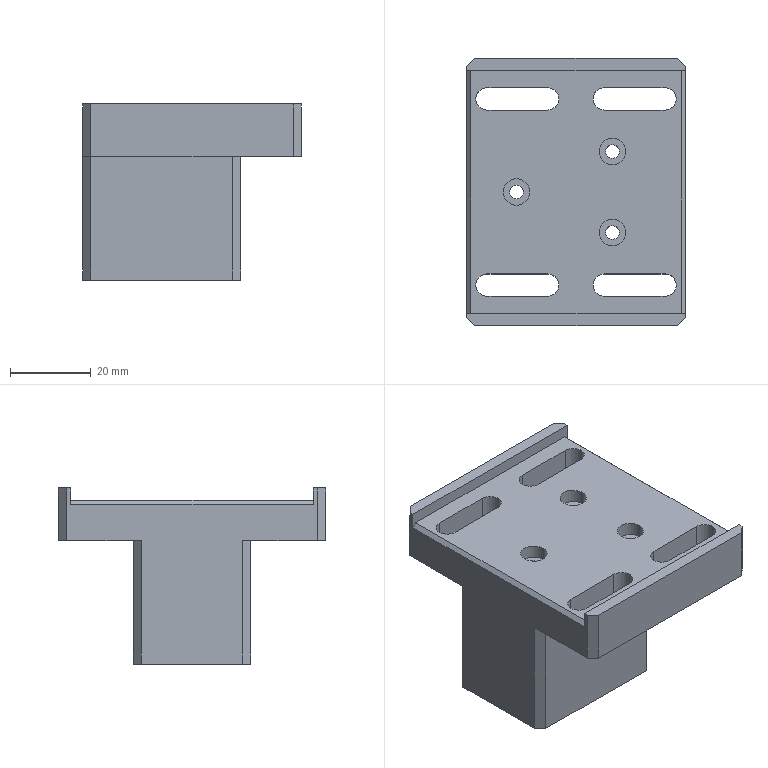Component | SolidWorks | ImagingSystem-1111-1_123456789-DL-OP20-ST12--003-1111-1 | 1 solid | 59 faces | box 54 x 66 x 43.5 mm | volume 65100 mm3 | plane 35 | cylinder 24 | commonest cylinder face diameters 5.5 x12 6.5 x6 3.4 x6 | material AL6061 Surface Hard Anodized
build123d program:
from build123d import *

# Parameters (mm, degrees)
SKETCH1_W                                       = 80
SKETCH1_H                                       = 60
BOSS_EXTRUDE1_DEPTH                             = 40.5
CUT_EXTRUDE1_DEPTH                              = 8
CUT_EXTRUDE5_DEPTH                              = 8
SKETCH12_W                                      = 80
SKETCH12_H                                      = 15.5
CUT_EXTRUDE9_DEPTH                              = 30.5
MOVE_FACE1_BY                                   = 45
SKETCH13_W                                      = 10
SKETCH13_H                                      = 60
BOSS_EXTRUDE2_DEPTH                             = 50
SKETCH14_W                                      = 35
SKETCH14_H                                      = 29
CUT_EXTRUDE10_DEPTH                             = 75.5
CHAMFER1_SIZE                                   = 2
SKETCH15_W                                      = 70.24
SKETCH15_H                                      = 79
CUT_EXTRUDE11_DEPTH                             = 100
MOVE_FACE2_BY                                   = 20
SKETCH16_W                                      = 20
SKETCH16_H                                      = 60
CUT_EXTRUDE12_DEPTH                             = 10
MOVE_FACE3_BY                                   = 3
MOVE_FACE3_2_BY                                 = 3
SKETCH18_W                                      = 54
SKETCH18_H                                      = 3
BOSS_EXTRUDE3_DEPTH                             = 3
CUT_EXTRUDE13_DEPTH                             = 20
CHAMFER5_SIZE                                   = 2
CHAMFER6_SIZE                                   = 1
MOVE_FACE4_BY                                   = 25
CHAMFER7_SIZE                                   = 2
M3_HEX_SOCKET_HEAD_CAP_SCREW_CBORE1_D           = 3.4
M3_HEX_SOCKET_HEAD_CAP_SCREW_CBORE1_CBORE_D     = 6.5
M3_HEX_SOCKET_HEAD_CAP_SCREW_CBORE1_CBORE_DEPTH = 3.4


with BuildPart() as part:
    # Sketch1 → Boss-Extrude1 (new body)
    with BuildSketch(Plane(origin=(45, 0, 0), x_dir=(0, 0, -1), z_dir=(1, 0, 0))):
        with Locations((10.458, -17.407)):
            Rectangle(SKETCH1_W, SKETCH1_H)
    extrude(amount=-BOSS_EXTRUDE1_DEPTH)

    # Sketch2 → Cut-Extrude1 (cut)
    with BuildSketch(Plane(origin=(45, 0, 0), x_dir=(0, 0, -1), z_dir=(1, 0, 0))):
        with BuildLine():
            Line((-4.542, -33.657), (-19.542, -33.657))
            ThreePointArc((-19.542, -33.657), (-24.292, -38.407), (-19.542, -43.157))
            Line((-19.542, -43.157), (-4.542, -43.157))
            ThreePointArc((-4.542, -43.157), (0.2076, -38.407), (-4.542, -33.657))
        make_face()
    extrude(amount=-CUT_EXTRUDE1_DEPTH, mode=Mode.SUBTRACT)

    # Sketch6 → Cut-Extrude5 (cut)
    with BuildSketch(Plane(origin=(45, 0, 0), x_dir=(0, 0, -1), z_dir=(1, 0, 0))):
        with BuildLine():
            Line((40.458, -33.657), (25.458, -33.657))
            ThreePointArc((25.458, -33.657), (20.708, -38.407), (25.458, -43.157))
            Line((25.458, -43.157), (40.458, -43.157))
            ThreePointArc((40.458, -43.157), (45.208, -38.407), (40.458, -33.657))
        make_face()
    extrude(amount=-CUT_EXTRUDE5_DEPTH, mode=Mode.SUBTRACT)

    # Sketch12 → Cut-Extrude9 (cut)
    with BuildSketch(Plane(origin=(45, 0, 0), x_dir=(0, 0, -1), z_dir=(1, 0, 0))):
        with Locations((10.458, 4.843)):
            Rectangle(SKETCH12_W, SKETCH12_H)
        with Locations((10.458, -39.657)):
            Rectangle(SKETCH12_W, SKETCH12_H)
    extrude(amount=-CUT_EXTRUDE9_DEPTH, mode=Mode.SUBTRACT)

    # Move Face1: a face moved outward by 45.0
    extrude(part.faces().sort_by_distance((45, -17.407, -10.458))[0], amount=MOVE_FACE1_BY, dir=(1, 0, 0))

    # Sketch13 → Boss-Extrude2 (add)
    with BuildSketch(Plane(origin=(0, 0, -50.458), x_dir=(-1, 0, 0), z_dir=(0, 0, -1))):
        with Locations((-9.5, -17.407)):
            Rectangle(SKETCH13_W, SKETCH13_H)
    extrude(amount=BOSS_EXTRUDE2_DEPTH)

    # Sketch14 → Cut-Extrude10 (cut)
    with BuildSketch(Plane(origin=(90, 0, 0), x_dir=(0, 0, -1), z_dir=(1, 0, 0))):
        with Locations((-12.042, -17.407)):
            Rectangle(SKETCH14_W, SKETCH14_H)
    extrude(amount=-CUT_EXTRUDE10_DEPTH, mode=Mode.SUBTRACT)

    # Chamfer1
    chamfer1_edges = [part.edges().sort_by_distance(p)[0] for p in [
        (52.25, -2.907, -50.458),
        (52.25, -31.907, -50.458),
        (52.25, -31.907, -5.458),
        (52.25, -2.907, -5.458),
    ]]
    chamfer(chamfer1_edges, length=CHAMFER1_SIZE)

    # Sketch15 → Cut-Extrude11 (cut)
    with BuildSketch(Plane(origin=(90, 0, 0), x_dir=(0, 0, -1), z_dir=(1, 0, 0))):
        with Locations((79.578, -17.407)):
            Rectangle(SKETCH15_W, SKETCH15_H)
    extrude(amount=-CUT_EXTRUDE11_DEPTH, mode=Mode.SUBTRACT)

    # Move Face2: a face moved inward by 20.0
    extrude(part.faces().sort_by_distance((90, -17.407, -25.024))[0], amount=MOVE_FACE2_BY, dir=(-1, 0, 0), mode=Mode.SUBTRACT)

    # Sketch16 → Cut-Extrude12 (cut)
    with BuildSketch(Plane(origin=(14.5, 0, 0), x_dir=(0, 0, -1), z_dir=(1, 0, 0))):
        with Locations((-19.542, -17.407)):
            Rectangle(SKETCH16_W, SKETCH16_H)
    extrude(amount=-CUT_EXTRUDE12_DEPTH, mode=Mode.SUBTRACT)

    # Move Face3: a face moved outward by 3.0
    extrude(part.faces().sort_by_distance((9.5, 12.593, -17.458))[0], amount=MOVE_FACE3_BY, dir=(0, 1, 0))

    # Move Face3 2: a face moved outward by 3.0
    extrude(part.faces().sort_by_distance((9.5, -47.407, -17.458))[0], amount=MOVE_FACE3_2_BY, dir=(0, -1, 0))

    # Sketch18 → Boss-Extrude3 (add)
    with BuildSketch(Plane.ZY.offset(-4.5)):
        with Locations((-17.458, 14.093)):
            Rectangle(SKETCH18_W, SKETCH18_H)
        with Locations((-17.458, -48.907)):
            Rectangle(SKETCH18_W, SKETCH18_H)
    extrude(amount=BOSS_EXTRUDE3_DEPTH)

    # Sketch19 → Cut-Extrude13 (cut)
    with BuildSketch(Plane(origin=(14.5, 0, 0), x_dir=(0, 0, -1), z_dir=(1, 0, 0))):
        with BuildLine():
            Line((-4.542, 8.343), (10.458, 8.343))
            ThreePointArc((10.458, 8.343), (13.208, 5.593), (10.458, 2.843))
            Line((10.458, 2.843), (-4.542, 2.843))
            ThreePointArc((-4.542, 2.843), (-7.292, 5.593), (-4.542, 8.343))
        make_face()
        with BuildLine():
            Line((24.458, 8.343), (39.458, 8.343))
            ThreePointArc((39.458, 8.343), (42.208, 5.593), (39.458, 2.843))
            Line((39.458, 2.843), (24.458, 2.843))
            ThreePointArc((24.458, 2.843), (21.708, 5.593), (24.458, 8.343))
        make_face()
        with BuildLine():
            Line((-4.542, -37.657), (10.458, -37.657))
            ThreePointArc((10.458, -37.657), (13.208, -40.407), (10.458, -43.157))
            Line((10.458, -43.157), (-4.542, -43.157))
            ThreePointArc((-4.542, -43.157), (-7.292, -40.407), (-4.542, -37.657))
        make_face()
        with BuildLine():
            Line((24.458, -37.657), (39.458, -37.657))
            ThreePointArc((39.458, -37.657), (42.208, -40.407), (39.458, -43.157))
            Line((39.458, -43.157), (24.458, -43.157))
            ThreePointArc((24.458, -43.157), (21.708, -40.407), (24.458, -37.657))
        make_face()
    extrude(amount=-CUT_EXTRUDE13_DEPTH, mode=Mode.SUBTRACT)

    # Chamfer5
    chamfer5_edges = [part.edges().sort_by_distance(p)[0] for p in [
        (8, -50.407, -44.458),
        (8, 15.593, -44.458),
        (8, 15.593, 9.542),
        (8, -50.407, 9.542),
    ]]
    chamfer(chamfer5_edges, length=CHAMFER5_SIZE)

    # Chamfer6
    chamfer6_edges = [part.edges().sort_by_distance(p)[0] for p in [
        (4.5, -17.407, 9.542),
        (4.5, -17.407, -44.458),
    ]]
    chamfer(chamfer6_edges, length=CHAMFER6_SIZE)

    # Move Face4: a face moved inward by 25.0
    extrude(part.faces().sort_by_distance((70, -17.407, -25.024))[0], amount=MOVE_FACE4_BY, dir=(-1, 0, 0), mode=Mode.SUBTRACT)

    # Chamfer7
    chamfer7_edges = [part.edges().sort_by_distance(p)[0] for p in [
        (29.75, -2.907, -44.458),
        (29.75, -31.907, -44.458),
    ]]
    chamfer(chamfer7_edges, length=CHAMFER7_SIZE)

    # M3 Hex Socket Head Cap Screw CBORE1 (through all)
    with Locations(Plane.ZY.offset(-4.5)):
        with Locations((-8.458, -27.407), (-8.458, -7.407), (-32.158, -17.407)):
            CounterBoreHole(M3_HEX_SOCKET_HEAD_CAP_SCREW_CBORE1_D / 2, M3_HEX_SOCKET_HEAD_CAP_SCREW_CBORE1_CBORE_D / 2, M3_HEX_SOCKET_HEAD_CAP_SCREW_CBORE1_CBORE_DEPTH)


solid = part.part

# Placed as in the assembly
solid = solid.moved(Location((27.142, -37.593, -15.5), (0, 90, 0)))